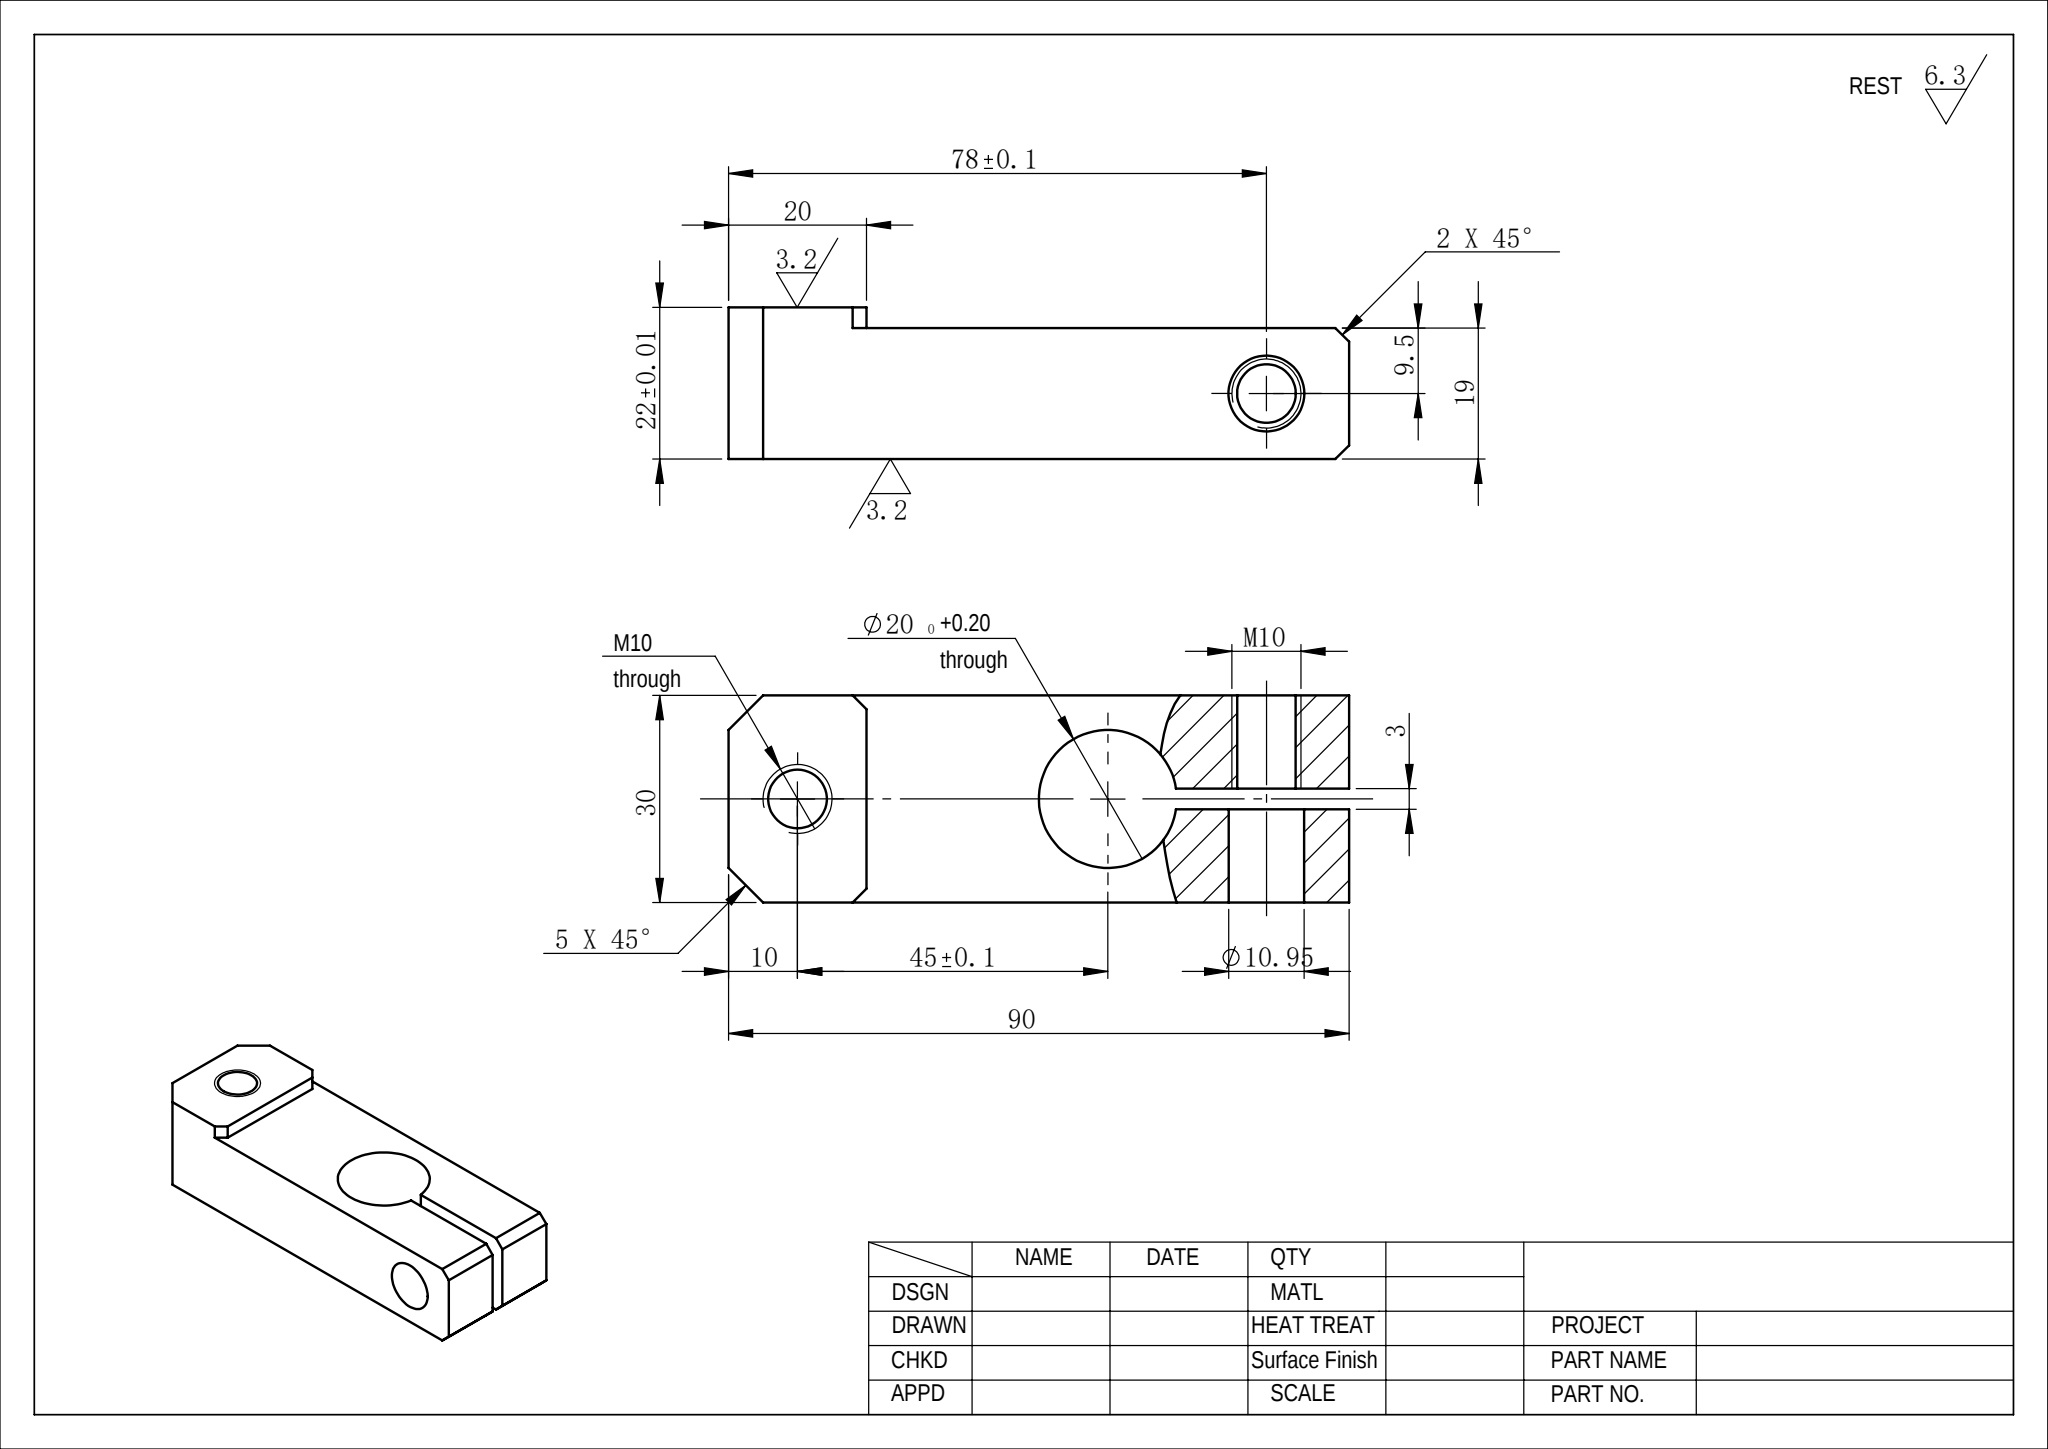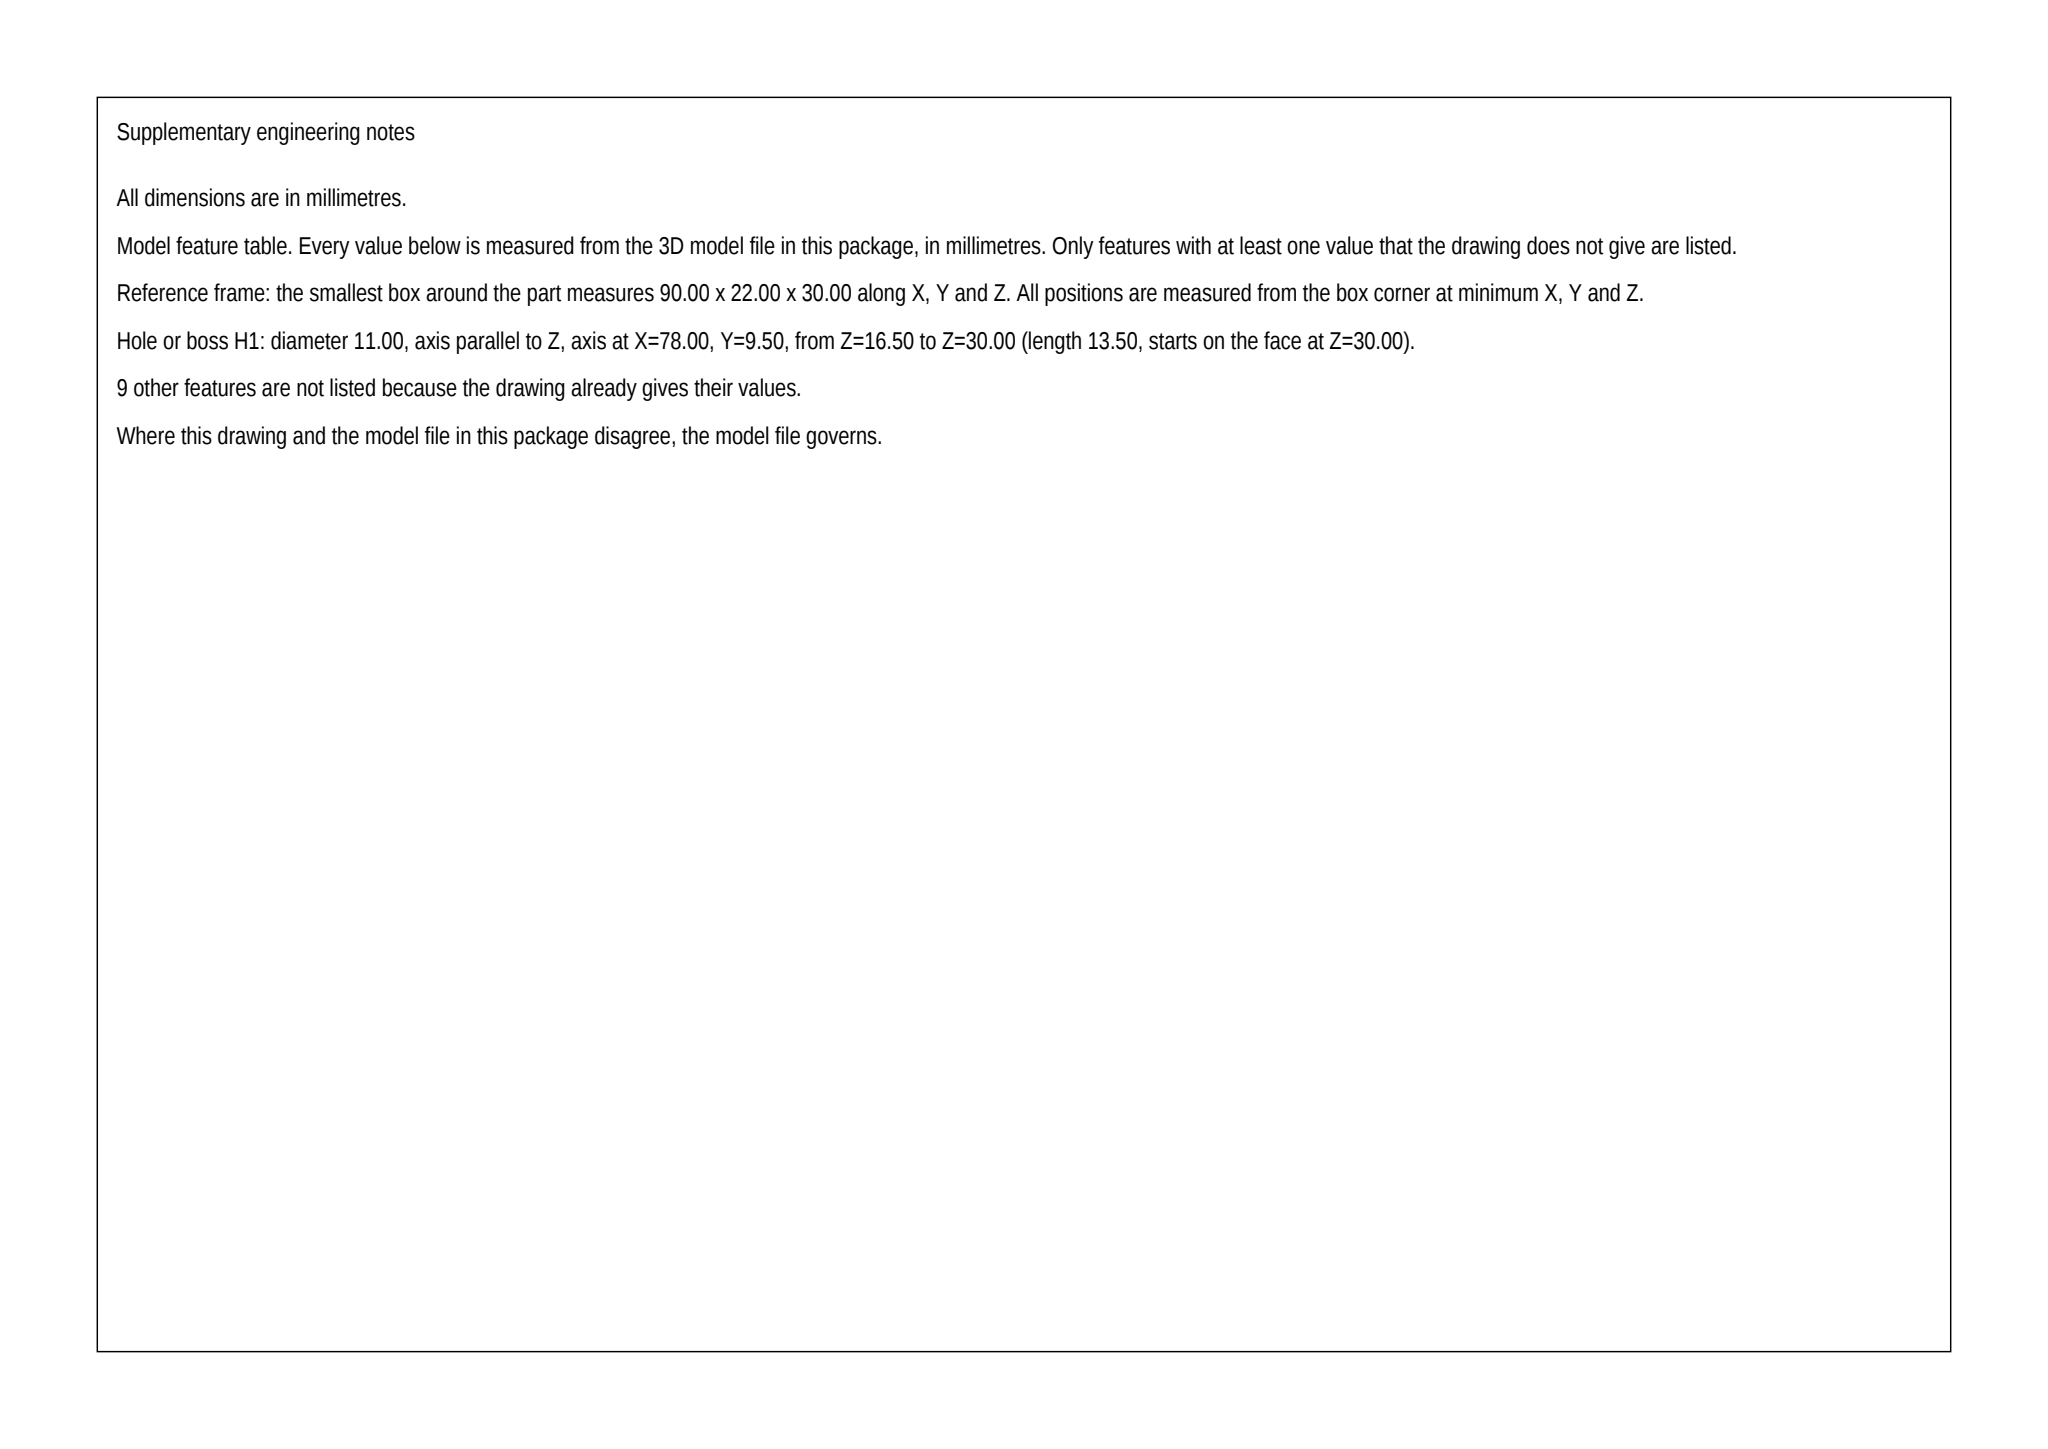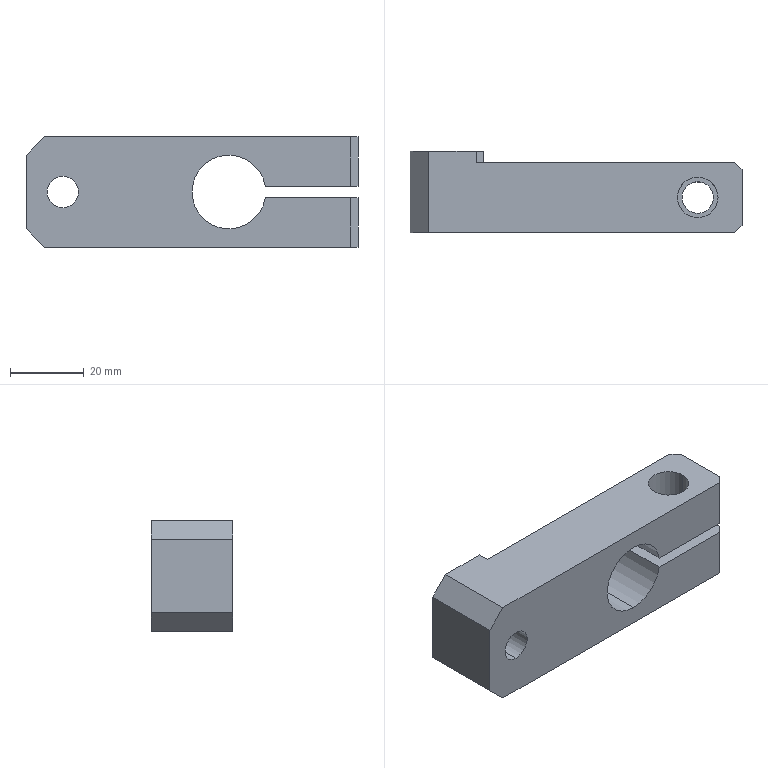Part | SolidWorks | mm | 1 solid | 28 faces | box 90 x 22 x 30 mm | volume 41736 mm3 | plane 19 | cylinder 9 | commonest cylinder face diameters 8.5 x4 20 x3 11 x2
build123d program:
from build123d import *

# Parameters (mm, degrees)
EXTRUDE1_DEPTH     = 30
M10_TAPPED_HOLE1_D = 8.5
SKETCH4_R          = 10
CUT_EXTRUDE1_DEPTH = 97.752
SKETCH5_R          = 5.5
CUT_EXTRUDE2_DEPTH = 15
SKETCH6_W          = 40.815
SKETCH6_H          = 3
CUT_EXTRUDE3_DEPTH = 97.752
M10_TAPPED_HOLE2_D = 8.5
CHAMFER1_SIZE      = 5
CHAMFER2_SIZE      = 2


with BuildPart() as part:
    # Sketch1 → Extrude1 (new body)
    with BuildSketch(Plane.XY):
        Polygon((0, 0), (0, 22), (20, 22), (20, 19), (90, 19), (90, 0), align=None)
    extrude(amount=EXTRUDE1_DEPTH)

    # M10 Tapped Hole1 (through all)
    with Locations(Plane(origin=(0, 22, 0), x_dir=(-1, 0, 0), z_dir=(0, 1, 0))):
        with Locations((-10, 15)):
            Hole(M10_TAPPED_HOLE1_D / 2)

    # Sketch4 → Cut-Extrude1 (cut, through all)
    with BuildSketch(Plane(origin=(0, 19, 0), x_dir=(1, 0, 0), z_dir=(0, 1, 0))):
        with Locations(Location((55, -15, 0), (0, 0, 270))):
            Circle(SKETCH4_R)
    extrude(amount=-CUT_EXTRUDE1_DEPTH, mode=Mode.SUBTRACT)

    # Sketch5 → Cut-Extrude2 (cut)
    with BuildSketch(Plane.XY.offset(30)):
        with Locations((78, 9.5)):
            Circle(SKETCH5_R)
    extrude(amount=-CUT_EXTRUDE2_DEPTH, mode=Mode.SUBTRACT)

    # Sketch6 → Cut-Extrude3 (cut, through all)
    with BuildSketch(Plane(origin=(0, 19, 0), x_dir=(1, 0, 0), z_dir=(0, 1, 0))):
        with Locations((72.3, -15)):
            Rectangle(SKETCH6_W, SKETCH6_H)
    extrude(amount=-CUT_EXTRUDE3_DEPTH, mode=Mode.SUBTRACT)

    # M10 Tapped Hole2 (through all)
    with Locations(Plane.XY.offset(13.5)):
        with Locations((78, 9.5)):
            Hole(M10_TAPPED_HOLE2_D / 2)

    # Chamfer1
    chamfer1_edges = [part.edges().sort_by_distance(p)[0] for p in [
        (0, 11, 30),
        (0, 11, 0),
    ]]
    chamfer(chamfer1_edges, length=CHAMFER1_SIZE)

    # Chamfer2
    chamfer2_edges = [part.edges().sort_by_distance(p)[0] for p in [
        (90, 19, 23.25),
        (90, 0, 23.25),
        (20, 20.5, 30),
        (90, 19, 6.75),
        (90, 0, 6.75),
        (20, 20.5, 0),
    ]]
    chamfer(chamfer2_edges, length=CHAMFER2_SIZE)


solid = part.part
STEP:
#1=CARTESIAN_POINT('',(73.75,9.5,0.));
#2=VERTEX_POINT('',#1);
#3=CARTESIAN_POINT('',(82.25,9.5,0.));
#4=VERTEX_POINT('',#3);
#5=CARTESIAN_POINT('',(78.,9.5,0.));
#6=DIRECTION('',(0.,0.,1.));
#7=DIRECTION('',(1.,0.,0.));
#8=AXIS2_PLACEMENT_3D('',#5,#6,#7);
#9=CIRCLE('',#8,4.25);
#10=EDGE_CURVE('',#2,#4,#9,.T.);
#11=ORIENTED_EDGE('',*,*,#10,.F.);
#12=CARTESIAN_POINT('',(73.75,9.5,13.5));
#13=VERTEX_POINT('',#12);
#14=CARTESIAN_POINT('',(73.75,9.5,13.5));
#15=DIRECTION('',(0.,0.,1.));
#16=VECTOR('',#15,1000.);
#17=LINE('',#14,#16);
#18=EDGE_CURVE('',#2,#13,#17,.T.);
#19=ORIENTED_EDGE('',*,*,#18,.T.);
#20=CARTESIAN_POINT('',(82.25,9.5,13.5));
#21=VERTEX_POINT('',#20);
#22=CARTESIAN_POINT('',(78.,9.5,13.5));
#23=DIRECTION('',(0.,0.,1.));
#24=DIRECTION('',(1.,0.,0.));
#25=AXIS2_PLACEMENT_3D('',#22,#23,#24);
#26=CIRCLE('',#25,4.25);
#27=EDGE_CURVE('',#13,#21,#26,.T.);
#28=ORIENTED_EDGE('',*,*,#27,.T.);
#29=CARTESIAN_POINT('',(82.25,9.5,13.5));
#30=DIRECTION('',(0.,0.,1.));
#31=VECTOR('',#30,1000.);
#32=LINE('',#29,#31);
#33=EDGE_CURVE('',#4,#21,#32,.T.);
#34=ORIENTED_EDGE('',*,*,#33,.F.);
#35=EDGE_LOOP('',(#11,#19,#28,#34));
#36=FACE_OUTER_BOUND('',#35,.T.);
#37=CARTESIAN_POINT('',(78.,9.5,13.5));
#38=DIRECTION('',(0.,0.,1.));
#39=DIRECTION('',(1.,0.,0.));
#40=AXIS2_PLACEMENT_3D('',#37,#38,#39);
#41=CYLINDRICAL_SURFACE('',#40,4.25);
#42=ADVANCED_FACE('',(#36),#41,.F.);
#43=CARTESIAN_POINT('',(83.5,9.5,16.5));
#44=VERTEX_POINT('',#43);
#45=CARTESIAN_POINT('',(72.5,9.5,16.5));
#46=VERTEX_POINT('',#45);
#47=CARTESIAN_POINT('',(78.,9.5,16.5));
#48=DIRECTION('',(0.,0.,-1.));
#49=DIRECTION('',(1.,0.,0.));
#50=AXIS2_PLACEMENT_3D('',#47,#48,#49);
#51=CIRCLE('',#50,5.5);
#52=EDGE_CURVE('',#44,#46,#51,.T.);
#53=ORIENTED_EDGE('',*,*,#52,.T.);
#54=CARTESIAN_POINT('',(72.5,9.5,30.));
#55=VERTEX_POINT('',#54);
#56=CARTESIAN_POINT('',(72.5,9.5,15.));
#57=DIRECTION('',(0.,0.,1.));
#58=VECTOR('',#57,1000.);
#59=LINE('',#56,#58);
#60=EDGE_CURVE('',#46,#55,#59,.T.);
#61=ORIENTED_EDGE('',*,*,#60,.T.);
#62=CARTESIAN_POINT('',(83.5,9.5,30.));
#63=VERTEX_POINT('',#62);
#64=CARTESIAN_POINT('',(78.,9.5,30.));
#65=DIRECTION('',(0.,0.,1.));
#66=DIRECTION('',(1.,0.,0.));
#67=AXIS2_PLACEMENT_3D('',#64,#65,#66);
#68=CIRCLE('',#67,5.5);
#69=EDGE_CURVE('',#55,#63,#68,.T.);
#70=ORIENTED_EDGE('',*,*,#69,.T.);
#71=CARTESIAN_POINT('',(83.5,9.5,15.));
#72=DIRECTION('',(0.,0.,1.));
#73=VECTOR('',#72,1000.);
#74=LINE('',#71,#73);
#75=EDGE_CURVE('',#44,#63,#74,.T.);
#76=ORIENTED_EDGE('',*,*,#75,.F.);
#77=EDGE_LOOP('',(#53,#61,#70,#76));
#78=FACE_OUTER_BOUND('',#77,.T.);
#79=CARTESIAN_POINT('',(78.,9.5,15.));
#80=DIRECTION('',(0.,0.,1.));
#81=DIRECTION('',(1.,0.,0.));
#82=AXIS2_PLACEMENT_3D('',#79,#80,#81);
#83=CYLINDRICAL_SURFACE('',#82,5.5);
#84=ADVANCED_FACE('',(#78),#83,.F.);
#85=CARTESIAN_POINT('',(55.,0.,5.));
#86=VERTEX_POINT('',#85);
#87=CARTESIAN_POINT('',(55.,0.,25.));
#88=VERTEX_POINT('',#87);
#89=CARTESIAN_POINT('',(55.,0.,15.));
#90=DIRECTION('',(0.,1.,0.));
#91=DIRECTION('',(0.,0.,1.));
#92=AXIS2_PLACEMENT_3D('',#89,#90,#91);
#93=CIRCLE('',#92,10.);
#94=EDGE_CURVE('',#86,#88,#93,.T.);
#95=ORIENTED_EDGE('',*,*,#94,.F.);
#96=CARTESIAN_POINT('',(55.,19.,5.));
#97=VERTEX_POINT('',#96);
#98=CARTESIAN_POINT('',(55.,0.,5.));
#99=DIRECTION('',(0.,1.,0.));
#100=VECTOR('',#99,1000.);
#101=LINE('',#98,#100);
#102=EDGE_CURVE('',#86,#97,#101,.T.);
#103=ORIENTED_EDGE('',*,*,#102,.T.);
#104=CARTESIAN_POINT('',(55.,19.,25.));
#105=VERTEX_POINT('',#104);
#106=CARTESIAN_POINT('',(55.,19.,15.));
#107=DIRECTION('',(0.,1.,0.));
#108=DIRECTION('',(0.,0.,1.));
#109=AXIS2_PLACEMENT_3D('',#106,#107,#108);
#110=CIRCLE('',#109,10.);
#111=EDGE_CURVE('',#97,#105,#110,.T.);
#112=ORIENTED_EDGE('',*,*,#111,.T.);
#113=CARTESIAN_POINT('',(55.,0.,25.));
#114=DIRECTION('',(0.,1.,0.));
#115=VECTOR('',#114,1000.);
#116=LINE('',#113,#115);
#117=EDGE_CURVE('',#88,#105,#116,.T.);
#118=ORIENTED_EDGE('',*,*,#117,.F.);
#119=EDGE_LOOP('',(#95,#103,#112,#118));
#120=FACE_OUTER_BOUND('',#119,.T.);
#121=CARTESIAN_POINT('',(55.,0.,15.));
#122=DIRECTION('',(0.,1.,0.));
#123=DIRECTION('',(0.,0.,1.));
#124=AXIS2_PLACEMENT_3D('',#121,#122,#123);
#125=CYLINDRICAL_SURFACE('',#124,10.);
#126=ADVANCED_FACE('',(#120),#125,.F.);
#127=CARTESIAN_POINT('',(64.887,0.,16.5));
#128=VERTEX_POINT('',#127);
#129=CARTESIAN_POINT('',(55.,0.,15.));
#130=DIRECTION('',(0.,1.,0.));
#131=DIRECTION('',(0.,0.,1.));
#132=AXIS2_PLACEMENT_3D('',#129,#130,#131);
#133=CIRCLE('',#132,10.);
#134=EDGE_CURVE('',#88,#128,#133,.T.);
#135=ORIENTED_EDGE('',*,*,#134,.F.);
#136=ORIENTED_EDGE('',*,*,#117,.T.);
#137=CARTESIAN_POINT('',(64.887,19.,16.5));
#138=VERTEX_POINT('',#137);
#139=CARTESIAN_POINT('',(55.,19.,15.));
#140=DIRECTION('',(0.,1.,0.));
#141=DIRECTION('',(0.,0.,1.));
#142=AXIS2_PLACEMENT_3D('',#139,#140,#141);
#143=CIRCLE('',#142,10.);
#144=EDGE_CURVE('',#105,#138,#143,.T.);
#145=ORIENTED_EDGE('',*,*,#144,.T.);
#146=CARTESIAN_POINT('',(64.887,0.,16.5));
#147=DIRECTION('',(0.,-1.,0.));
#148=VECTOR('',#147,1000.);
#149=LINE('',#146,#148);
#150=EDGE_CURVE('',#138,#128,#149,.T.);
#151=ORIENTED_EDGE('',*,*,#150,.T.);
#152=EDGE_LOOP('',(#135,#136,#145,#151));
#153=FACE_OUTER_BOUND('',#152,.T.);
#154=CARTESIAN_POINT('',(55.,0.,15.));
#155=DIRECTION('',(0.,1.,0.));
#156=DIRECTION('',(0.,0.,1.));
#157=AXIS2_PLACEMENT_3D('',#154,#155,#156);
#158=CYLINDRICAL_SURFACE('',#157,10.);
#159=ADVANCED_FACE('',(#153),#158,.F.);
#160=CARTESIAN_POINT('',(10.,0.,10.75));
#161=VERTEX_POINT('',#160);
#162=CARTESIAN_POINT('',(10.,0.,19.25));
#163=VERTEX_POINT('',#162);
#164=CARTESIAN_POINT('',(10.,0.,15.));
#165=DIRECTION('',(0.,1.,0.));
#166=DIRECTION('',(0.,0.,1.));
#167=AXIS2_PLACEMENT_3D('',#164,#165,#166);
#168=CIRCLE('',#167,4.25);
#169=EDGE_CURVE('',#161,#163,#168,.T.);
#170=ORIENTED_EDGE('',*,*,#169,.F.);
#171=CARTESIAN_POINT('',(10.,22.,10.75));
#172=VERTEX_POINT('',#171);
#173=CARTESIAN_POINT('',(10.,22.,10.75));
#174=DIRECTION('',(0.,1.,0.));
#175=VECTOR('',#174,1000.);
#176=LINE('',#173,#175);
#177=EDGE_CURVE('',#161,#172,#176,.T.);
#178=ORIENTED_EDGE('',*,*,#177,.T.);
#179=CARTESIAN_POINT('',(10.,22.,19.25));
#180=VERTEX_POINT('',#179);
#181=CARTESIAN_POINT('',(10.,22.,15.));
#182=DIRECTION('',(0.,1.,0.));
#183=DIRECTION('',(0.,0.,1.));
#184=AXIS2_PLACEMENT_3D('',#181,#182,#183);
#185=CIRCLE('',#184,4.25);
#186=EDGE_CURVE('',#172,#180,#185,.T.);
#187=ORIENTED_EDGE('',*,*,#186,.T.);
#188=CARTESIAN_POINT('',(10.,22.,19.25));
#189=DIRECTION('',(0.,1.,0.));
#190=VECTOR('',#189,1000.);
#191=LINE('',#188,#190);
#192=EDGE_CURVE('',#163,#180,#191,.T.);
#193=ORIENTED_EDGE('',*,*,#192,.F.);
#194=EDGE_LOOP('',(#170,#178,#187,#193));
#195=FACE_OUTER_BOUND('',#194,.T.);
#196=CARTESIAN_POINT('',(10.,22.,15.));
#197=DIRECTION('',(0.,1.,0.));
#198=DIRECTION('',(0.,0.,1.));
#199=AXIS2_PLACEMENT_3D('',#196,#197,#198);
#200=CYLINDRICAL_SURFACE('',#199,4.25);
#201=ADVANCED_FACE('',(#195),#200,.F.);
#202=CARTESIAN_POINT('',(18.,22.,0.));
#203=VERTEX_POINT('',#202);
#204=CARTESIAN_POINT('',(5.,22.,-0.));
#205=VERTEX_POINT('',#204);
#206=CARTESIAN_POINT('',(0.,22.,0.));
#207=DIRECTION('',(-1.,0.,0.));
#208=VECTOR('',#207,1000.);
#209=LINE('',#206,#208);
#210=EDGE_CURVE('',#203,#205,#209,.T.);
#211=ORIENTED_EDGE('',*,*,#210,.F.);
#212=CARTESIAN_POINT('',(18.,19.,0.));
#213=VERTEX_POINT('',#212);
#214=CARTESIAN_POINT('',(18.,19.,0.));
#215=DIRECTION('',(0.,-1.,0.));
#216=VECTOR('',#215,1000.);
#217=LINE('',#214,#216);
#218=EDGE_CURVE('',#203,#213,#217,.T.);
#219=ORIENTED_EDGE('',*,*,#218,.T.);
#220=CARTESIAN_POINT('',(88.,19.,0.));
#221=VERTEX_POINT('',#220);
#222=CARTESIAN_POINT('',(20.,19.,0.));
#223=DIRECTION('',(-1.,0.,0.));
#224=VECTOR('',#223,1000.);
#225=LINE('',#222,#224);
#226=EDGE_CURVE('',#221,#213,#225,.T.);
#227=ORIENTED_EDGE('',*,*,#226,.F.);
#228=CARTESIAN_POINT('',(90.,17.,0.));
#229=VERTEX_POINT('',#228);
#230=CARTESIAN_POINT('',(53.5,53.5,0.));
#231=DIRECTION('',(0.7071,-0.7071,0.));
#232=VECTOR('',#231,1000.);
#233=LINE('',#230,#232);
#234=EDGE_CURVE('',#221,#229,#233,.T.);
#235=ORIENTED_EDGE('',*,*,#234,.T.);
#236=CARTESIAN_POINT('',(90.,2.,0.));
#237=VERTEX_POINT('',#236);
#238=CARTESIAN_POINT('',(90.,19.,0.));
#239=DIRECTION('',(0.,1.,0.));
#240=VECTOR('',#239,1000.);
#241=LINE('',#238,#240);
#242=EDGE_CURVE('',#237,#229,#241,.T.);
#243=ORIENTED_EDGE('',*,*,#242,.F.);
#244=CARTESIAN_POINT('',(88.,0.,0.));
#245=VERTEX_POINT('',#244);
#246=CARTESIAN_POINT('',(44.,-44.,0.));
#247=DIRECTION('',(-0.7071,-0.7071,0.));
#248=VECTOR('',#247,1000.);
#249=LINE('',#246,#248);
#250=EDGE_CURVE('',#237,#245,#249,.T.);
#251=ORIENTED_EDGE('',*,*,#250,.T.);
#252=CARTESIAN_POINT('',(5.,0.,0.));
#253=VERTEX_POINT('',#252);
#254=CARTESIAN_POINT('',(90.,0.,0.));
#255=DIRECTION('',(1.,0.,0.));
#256=VECTOR('',#255,1000.);
#257=LINE('',#254,#256);
#258=EDGE_CURVE('',#253,#245,#257,.T.);
#259=ORIENTED_EDGE('',*,*,#258,.F.);
#260=CARTESIAN_POINT('',(5.,22.,0.));
#261=DIRECTION('',(0.,1.,0.));
#262=VECTOR('',#261,1000.);
#263=LINE('',#260,#262);
#264=EDGE_CURVE('',#253,#205,#263,.T.);
#265=ORIENTED_EDGE('',*,*,#264,.T.);
#266=EDGE_LOOP('',(#211,#219,#227,#235,#243,#251,#259,#265));
#267=FACE_OUTER_BOUND('',#266,.T.);
#268=CARTESIAN_POINT('',(78.,9.5,0.));
#269=DIRECTION('',(0.,0.,1.));
#270=DIRECTION('',(1.,0.,0.));
#271=AXIS2_PLACEMENT_3D('',#268,#269,#270);
#272=CIRCLE('',#271,4.25);
#273=EDGE_CURVE('',#4,#2,#272,.T.);
#274=ORIENTED_EDGE('',*,*,#273,.T.);
#275=ORIENTED_EDGE('',*,*,#10,.T.);
#276=EDGE_LOOP('',(#274,#275));
#277=FACE_BOUND('',#276,.T.);
#278=CARTESIAN_POINT('',(0.,0.,0.));
#279=DIRECTION('',(0.,0.,-1.));
#280=DIRECTION('',(-1.,0.,0.));
#281=AXIS2_PLACEMENT_3D('',#278,#279,#280);
#282=PLANE('',#281);
#283=ADVANCED_FACE('',(#267,#277),#282,.T.);
#284=CARTESIAN_POINT('',(90.,17.,13.5));
#285=VERTEX_POINT('',#284);
#286=CARTESIAN_POINT('',(90.,2.,13.5));
#287=VERTEX_POINT('',#286);
#288=CARTESIAN_POINT('',(90.,19.,13.5));
#289=DIRECTION('',(0.,-1.,0.));
#290=VECTOR('',#289,1000.);
#291=LINE('',#288,#290);
#292=EDGE_CURVE('',#285,#287,#291,.T.);
#293=ORIENTED_EDGE('',*,*,#292,.T.);
#294=CARTESIAN_POINT('',(90.,2.,30.));
#295=DIRECTION('',(0.,0.,-1.));
#296=VECTOR('',#295,1000.);
#297=LINE('',#294,#296);
#298=EDGE_CURVE('',#287,#237,#297,.T.);
#299=ORIENTED_EDGE('',*,*,#298,.T.);
#300=ORIENTED_EDGE('',*,*,#242,.T.);
#301=CARTESIAN_POINT('',(90.,17.,30.));
#302=DIRECTION('',(0.,0.,1.));
#303=VECTOR('',#302,1000.);
#304=LINE('',#301,#303);
#305=EDGE_CURVE('',#229,#285,#304,.T.);
#306=ORIENTED_EDGE('',*,*,#305,.T.);
#307=EDGE_LOOP('',(#293,#299,#300,#306));
#308=FACE_OUTER_BOUND('',#307,.T.);
#309=CARTESIAN_POINT('',(90.,19.,30.));
#310=DIRECTION('',(-1.,0.,0.));
#311=DIRECTION('',(0.,0.,1.));
#312=AXIS2_PLACEMENT_3D('',#309,#310,#311);
#313=PLANE('',#312);
#314=ADVANCED_FACE('',(#308),#313,.F.);
#315=ORIENTED_EDGE('',*,*,#258,.T.);
#316=CARTESIAN_POINT('',(88.,-0.,13.5));
#317=VERTEX_POINT('',#316);
#318=CARTESIAN_POINT('',(88.,0.,30.));
#319=DIRECTION('',(0.,0.,1.));
#320=VECTOR('',#319,1000.);
#321=LINE('',#318,#320);
#322=EDGE_CURVE('',#245,#317,#321,.T.);
#323=ORIENTED_EDGE('',*,*,#322,.T.);
#324=CARTESIAN_POINT('',(64.887,0.,13.5));
#325=VERTEX_POINT('',#324);
#326=CARTESIAN_POINT('',(51.893,0.,13.5));
#327=DIRECTION('',(-1.,0.,0.));
#328=VECTOR('',#327,1000.);
#329=LINE('',#326,#328);
#330=EDGE_CURVE('',#317,#325,#329,.T.);
#331=ORIENTED_EDGE('',*,*,#330,.T.);
#332=CARTESIAN_POINT('',(55.,0.,15.));
#333=DIRECTION('',(0.,1.,0.));
#334=DIRECTION('',(0.,0.,1.));
#335=AXIS2_PLACEMENT_3D('',#332,#333,#334);
#336=CIRCLE('',#335,10.);
#337=EDGE_CURVE('',#325,#86,#336,.T.);
#338=ORIENTED_EDGE('',*,*,#337,.T.);
#339=ORIENTED_EDGE('',*,*,#94,.T.);
#340=ORIENTED_EDGE('',*,*,#134,.T.);
#341=CARTESIAN_POINT('',(88.,0.,16.5));
#342=VERTEX_POINT('',#341);
#343=CARTESIAN_POINT('',(51.893,0.,16.5));
#344=DIRECTION('',(1.,0.,0.));
#345=VECTOR('',#344,1000.);
#346=LINE('',#343,#345);
#347=EDGE_CURVE('',#128,#342,#346,.T.);
#348=ORIENTED_EDGE('',*,*,#347,.T.);
#349=CARTESIAN_POINT('',(88.,0.,30.));
#350=VERTEX_POINT('',#349);
#351=CARTESIAN_POINT('',(88.,0.,30.));
#352=DIRECTION('',(0.,0.,1.));
#353=VECTOR('',#352,1000.);
#354=LINE('',#351,#353);
#355=EDGE_CURVE('',#342,#350,#354,.T.);
#356=ORIENTED_EDGE('',*,*,#355,.T.);
#357=CARTESIAN_POINT('',(5.,0.,30.));
#358=VERTEX_POINT('',#357);
#359=CARTESIAN_POINT('',(90.,0.,30.));
#360=DIRECTION('',(1.,0.,0.));
#361=VECTOR('',#360,1000.);
#362=LINE('',#359,#361);
#363=EDGE_CURVE('',#358,#350,#362,.T.);
#364=ORIENTED_EDGE('',*,*,#363,.F.);
#365=CARTESIAN_POINT('',(0.,0.,25.));
#366=VERTEX_POINT('',#365);
#367=CARTESIAN_POINT('',(5.,0.,30.));
#368=DIRECTION('',(-0.7071,-0.,-0.7071));
#369=VECTOR('',#368,1000.);
#370=LINE('',#367,#369);
#371=EDGE_CURVE('',#358,#366,#370,.T.);
#372=ORIENTED_EDGE('',*,*,#371,.T.);
#373=CARTESIAN_POINT('',(0.,0.,5.));
#374=VERTEX_POINT('',#373);
#375=CARTESIAN_POINT('',(0.,0.,30.));
#376=DIRECTION('',(0.,0.,-1.));
#377=VECTOR('',#376,1000.);
#378=LINE('',#375,#377);
#379=EDGE_CURVE('',#366,#374,#378,.T.);
#380=ORIENTED_EDGE('',*,*,#379,.T.);
#381=CARTESIAN_POINT('',(0.,0.,5.));
#382=DIRECTION('',(0.7071,0.,-0.7071));
#383=VECTOR('',#382,1000.);
#384=LINE('',#381,#383);
#385=EDGE_CURVE('',#374,#253,#384,.T.);
#386=ORIENTED_EDGE('',*,*,#385,.T.);
#387=EDGE_LOOP('',(#315,#323,#331,#338,#339,#340,#348,#356,#364,#372,#380,#386));
#388=FACE_OUTER_BOUND('',#387,.T.);
#389=CARTESIAN_POINT('',(10.,0.,15.));
#390=DIRECTION('',(0.,1.,0.));
#391=DIRECTION('',(0.,0.,1.));
#392=AXIS2_PLACEMENT_3D('',#389,#390,#391);
#393=CIRCLE('',#392,4.25);
#394=EDGE_CURVE('',#163,#161,#393,.T.);
#395=ORIENTED_EDGE('',*,*,#394,.T.);
#396=ORIENTED_EDGE('',*,*,#169,.T.);
#397=EDGE_LOOP('',(#395,#396));
#398=FACE_BOUND('',#397,.T.);
#399=CARTESIAN_POINT('',(90.,0.,30.));
#400=DIRECTION('',(-0.,1.,0.));
#401=DIRECTION('',(-1.,-0.,0.));
#402=AXIS2_PLACEMENT_3D('',#399,#400,#401);
#403=PLANE('',#402);
#404=ADVANCED_FACE('',(#388,#398),#403,.F.);
#405=CARTESIAN_POINT('',(90.,2.,30.));
#406=VERTEX_POINT('',#405);
#407=CARTESIAN_POINT('',(90.,17.,30.));
#408=VERTEX_POINT('',#407);
#409=CARTESIAN_POINT('',(90.,19.,30.));
#410=DIRECTION('',(0.,1.,0.));
#411=VECTOR('',#410,1000.);
#412=LINE('',#409,#411);
#413=EDGE_CURVE('',#406,#408,#412,.T.);
#414=ORIENTED_EDGE('',*,*,#413,.F.);
#415=CARTESIAN_POINT('',(90.,2.,16.5));
#416=VERTEX_POINT('',#415);
#417=CARTESIAN_POINT('',(90.,2.,30.));
#418=DIRECTION('',(0.,0.,-1.));
#419=VECTOR('',#418,1000.);
#420=LINE('',#417,#419);
#421=EDGE_CURVE('',#406,#416,#420,.T.);
#422=ORIENTED_EDGE('',*,*,#421,.T.);
#423=CARTESIAN_POINT('',(90.,17.,16.5));
#424=VERTEX_POINT('',#423);
#425=CARTESIAN_POINT('',(90.,19.,16.5));
#426=DIRECTION('',(0.,1.,0.));
#427=VECTOR('',#426,1000.);
#428=LINE('',#425,#427);
#429=EDGE_CURVE('',#416,#424,#428,.T.);
#430=ORIENTED_EDGE('',*,*,#429,.T.);
#431=CARTESIAN_POINT('',(90.,17.,30.));
#432=DIRECTION('',(0.,0.,1.));
#433=VECTOR('',#432,1000.);
#434=LINE('',#431,#433);
#435=EDGE_CURVE('',#424,#408,#434,.T.);
#436=ORIENTED_EDGE('',*,*,#435,.T.);
#437=EDGE_LOOP('',(#414,#422,#430,#436));
#438=FACE_OUTER_BOUND('',#437,.T.);
#439=CARTESIAN_POINT('',(90.,19.,30.));
#440=DIRECTION('',(-1.,0.,0.));
#441=DIRECTION('',(0.,0.,1.));
#442=AXIS2_PLACEMENT_3D('',#439,#440,#441);
#443=PLANE('',#442);
#444=ADVANCED_FACE('',(#438),#443,.F.);
#445=CARTESIAN_POINT('',(88.,19.,13.5));
#446=VERTEX_POINT('',#445);
#447=CARTESIAN_POINT('',(64.887,19.,13.5));
#448=VERTEX_POINT('',#447);
#449=CARTESIAN_POINT('',(51.893,19.,13.5));
#450=DIRECTION('',(-1.,0.,0.));
#451=VECTOR('',#450,1000.);
#452=LINE('',#449,#451);
#453=EDGE_CURVE('',#446,#448,#452,.T.);
#454=ORIENTED_EDGE('',*,*,#453,.F.);
#455=CARTESIAN_POINT('',(88.,19.,30.));
#456=DIRECTION('',(0.,0.,-1.));
#457=VECTOR('',#456,1000.);
#458=LINE('',#455,#457);
#459=EDGE_CURVE('',#446,#221,#458,.T.);
#460=ORIENTED_EDGE('',*,*,#459,.T.);
#461=ORIENTED_EDGE('',*,*,#226,.T.);
#462=CARTESIAN_POINT('',(20.,19.,2.));
#463=VERTEX_POINT('',#462);
#464=CARTESIAN_POINT('',(34.,19.,16.));
#465=DIRECTION('',(0.7071,0.,0.7071));
#466=VECTOR('',#465,1000.);
#467=LINE('',#464,#466);
#468=EDGE_CURVE('',#213,#463,#467,.T.);
#469=ORIENTED_EDGE('',*,*,#468,.T.);
#470=CARTESIAN_POINT('',(20.,19.,28.));
#471=VERTEX_POINT('',#470);
#472=CARTESIAN_POINT('',(20.,19.,30.));
#473=DIRECTION('',(0.,0.,-1.));
#474=VECTOR('',#473,1000.);
#475=LINE('',#472,#474);
#476=EDGE_CURVE('',#471,#463,#475,.T.);
#477=ORIENTED_EDGE('',*,*,#476,.F.);
#478=CARTESIAN_POINT('',(18.,19.,30.));
#479=VERTEX_POINT('',#478);
#480=CARTESIAN_POINT('',(19.,19.,29.));
#481=DIRECTION('',(-0.7071,0.,0.7071));
#482=VECTOR('',#481,1000.);
#483=LINE('',#480,#482);
#484=EDGE_CURVE('',#471,#479,#483,.T.);
#485=ORIENTED_EDGE('',*,*,#484,.T.);
#486=CARTESIAN_POINT('',(88.,19.,30.));
#487=VERTEX_POINT('',#486);
#488=CARTESIAN_POINT('',(20.,19.,30.));
#489=DIRECTION('',(-1.,0.,0.));
#490=VECTOR('',#489,1000.);
#491=LINE('',#488,#490);
#492=EDGE_CURVE('',#487,#479,#491,.T.);
#493=ORIENTED_EDGE('',*,*,#492,.F.);
#494=CARTESIAN_POINT('',(88.,19.,16.5));
#495=VERTEX_POINT('',#494);
#496=CARTESIAN_POINT('',(88.,19.,30.));
#497=DIRECTION('',(0.,0.,-1.));
#498=VECTOR('',#497,1000.);
#499=LINE('',#496,#498);
#500=EDGE_CURVE('',#487,#495,#499,.T.);
#501=ORIENTED_EDGE('',*,*,#500,.T.);
#502=CARTESIAN_POINT('',(51.893,19.,16.5));
#503=DIRECTION('',(1.,0.,0.));
#504=VECTOR('',#503,1000.);
#505=LINE('',#502,#504);
#506=EDGE_CURVE('',#138,#495,#505,.T.);
#507=ORIENTED_EDGE('',*,*,#506,.F.);
#508=ORIENTED_EDGE('',*,*,#144,.F.);
#509=ORIENTED_EDGE('',*,*,#111,.F.);
#510=CARTESIAN_POINT('',(55.,19.,15.));
#511=DIRECTION('',(0.,1.,0.));
#512=DIRECTION('',(0.,0.,1.));
#513=AXIS2_PLACEMENT_3D('',#510,#511,#512);
#514=CIRCLE('',#513,10.);
#515=EDGE_CURVE('',#448,#97,#514,.T.);
#516=ORIENTED_EDGE('',*,*,#515,.F.);
#517=EDGE_LOOP('',(#454,#460,#461,#469,#477,#485,#493,#501,#507,#508,#509,#516));
#518=FACE_OUTER_BOUND('',#517,.T.);
#519=CARTESIAN_POINT('',(20.,19.,30.));
#520=DIRECTION('',(0.,-1.,0.));
#521=DIRECTION('',(0.,0.,-1.));
#522=AXIS2_PLACEMENT_3D('',#519,#520,#521);
#523=PLANE('',#522);
#524=ADVANCED_FACE('',(#518),#523,.F.);
#525=ORIENTED_EDGE('',*,*,#476,.T.);
#526=CARTESIAN_POINT('',(20.,22.,2.));
#527=VERTEX_POINT('',#526);
#528=CARTESIAN_POINT('',(20.,22.,2.));
#529=DIRECTION('',(0.,1.,0.));
#530=VECTOR('',#529,1000.);
#531=LINE('',#528,#530);
#532=EDGE_CURVE('',#463,#527,#531,.T.);
#533=ORIENTED_EDGE('',*,*,#532,.T.);
#534=CARTESIAN_POINT('',(20.,22.,28.));
#535=VERTEX_POINT('',#534);
#536=CARTESIAN_POINT('',(20.,22.,30.));
#537=DIRECTION('',(0.,0.,-1.));
#538=VECTOR('',#537,1000.);
#539=LINE('',#536,#538);
#540=EDGE_CURVE('',#535,#527,#539,.T.);
#541=ORIENTED_EDGE('',*,*,#540,.F.);
#542=CARTESIAN_POINT('',(20.,22.,28.));
#543=DIRECTION('',(0.,-1.,0.));
#544=VECTOR('',#543,1000.);
#545=LINE('',#542,#544);
#546=EDGE_CURVE('',#535,#471,#545,.T.);
#547=ORIENTED_EDGE('',*,*,#546,.T.);
#548=EDGE_LOOP('',(#525,#533,#541,#547));
#549=FACE_OUTER_BOUND('',#548,.T.);
#550=CARTESIAN_POINT('',(20.,22.,30.));
#551=DIRECTION('',(-1.,0.,0.));
#552=DIRECTION('',(0.,0.,1.));
#553=AXIS2_PLACEMENT_3D('',#550,#551,#552);
#554=PLANE('',#553);
#555=ADVANCED_FACE('',(#549),#554,.F.);
#556=CARTESIAN_POINT('',(10.,22.,15.));
#557=DIRECTION('',(0.,1.,0.));
#558=DIRECTION('',(0.,0.,1.));
#559=AXIS2_PLACEMENT_3D('',#556,#557,#558);
#560=CIRCLE('',#559,4.25);
#561=EDGE_CURVE('',#180,#172,#560,.T.);
#562=ORIENTED_EDGE('',*,*,#561,.F.);
#563=ORIENTED_EDGE('',*,*,#186,.F.);
#564=EDGE_LOOP('',(#562,#563));
#565=FACE_BOUND('',#564,.T.);
#566=ORIENTED_EDGE('',*,*,#540,.T.);
#567=CARTESIAN_POINT('',(20.,22.,2.));
#568=DIRECTION('',(-0.7071,0.,-0.7071));
#569=VECTOR('',#568,1000.);
#570=LINE('',#567,#569);
#571=EDGE_CURVE('',#527,#203,#570,.T.);
#572=ORIENTED_EDGE('',*,*,#571,.T.);
#573=ORIENTED_EDGE('',*,*,#210,.T.);
#574=CARTESIAN_POINT('',(-0.,22.,5.));
#575=VERTEX_POINT('',#574);
#576=CARTESIAN_POINT('',(0.,22.,5.));
#577=DIRECTION('',(-0.7071,0.,0.7071));
#578=VECTOR('',#577,1000.);
#579=LINE('',#576,#578);
#580=EDGE_CURVE('',#205,#575,#579,.T.);
#581=ORIENTED_EDGE('',*,*,#580,.T.);
#582=CARTESIAN_POINT('',(0.,22.,25.));
#583=VERTEX_POINT('',#582);
#584=CARTESIAN_POINT('',(0.,22.,30.));
#585=DIRECTION('',(0.,0.,-1.));
#586=VECTOR('',#585,1000.);
#587=LINE('',#584,#586);
#588=EDGE_CURVE('',#583,#575,#587,.T.);
#589=ORIENTED_EDGE('',*,*,#588,.F.);
#590=CARTESIAN_POINT('',(5.,22.,30.));
#591=VERTEX_POINT('',#590);
#592=CARTESIAN_POINT('',(5.,22.,30.));
#593=DIRECTION('',(0.7071,0.,0.7071));
#594=VECTOR('',#593,1000.);
#595=LINE('',#592,#594);
#596=EDGE_CURVE('',#583,#591,#595,.T.);
#597=ORIENTED_EDGE('',*,*,#596,.T.);
#598=CARTESIAN_POINT('',(18.,22.,30.));
#599=VERTEX_POINT('',#598);
#600=CARTESIAN_POINT('',(0.,22.,30.));
#601=DIRECTION('',(-1.,0.,0.));
#602=VECTOR('',#601,1000.);
#603=LINE('',#600,#602);
#604=EDGE_CURVE('',#599,#591,#603,.T.);
#605=ORIENTED_EDGE('',*,*,#604,.F.);
#606=CARTESIAN_POINT('',(18.,22.,30.));
#607=DIRECTION('',(0.7071,0.,-0.7071));
#608=VECTOR('',#607,1000.);
#609=LINE('',#606,#608);
#610=EDGE_CURVE('',#599,#535,#609,.T.);
#611=ORIENTED_EDGE('',*,*,#610,.T.);
#612=EDGE_LOOP('',(#566,#572,#573,#581,#589,#597,#605,#611));
#613=FACE_OUTER_BOUND('',#612,.T.);
#614=CARTESIAN_POINT('',(0.,22.,30.));
#615=DIRECTION('',(0.,-1.,0.));
#616=DIRECTION('',(0.,0.,-1.));
#617=AXIS2_PLACEMENT_3D('',#614,#615,#616);
#618=PLANE('',#617);
#619=ADVANCED_FACE('',(#565,#613),#618,.F.);
#620=ORIENTED_EDGE('',*,*,#588,.T.);
#621=CARTESIAN_POINT('',(0.,0.,5.));
#622=DIRECTION('',(0.,-1.,0.));
#623=VECTOR('',#622,1000.);
#624=LINE('',#621,#623);
#625=EDGE_CURVE('',#575,#374,#624,.T.);
#626=ORIENTED_EDGE('',*,*,#625,.T.);
#627=ORIENTED_EDGE('',*,*,#379,.F.);
#628=CARTESIAN_POINT('',(0.,0.,25.));
#629=DIRECTION('',(0.,1.,0.));
#630=VECTOR('',#629,1000.);
#631=LINE('',#628,#630);
#632=EDGE_CURVE('',#366,#583,#631,.T.);
#633=ORIENTED_EDGE('',*,*,#632,.T.);
#634=EDGE_LOOP('',(#620,#626,#627,#633));
#635=FACE_OUTER_BOUND('',#634,.T.);
#636=CARTESIAN_POINT('',(0.,0.,30.));
#637=DIRECTION('',(1.,0.,0.));
#638=DIRECTION('',(0.,0.,-1.));
#639=AXIS2_PLACEMENT_3D('',#636,#637,#638);
#640=PLANE('',#639);
#641=ADVANCED_FACE('',(#635),#640,.F.);
#642=CARTESIAN_POINT('',(78.,9.5,30.));
#643=DIRECTION('',(0.,0.,1.));
#644=DIRECTION('',(1.,0.,0.));
#645=AXIS2_PLACEMENT_3D('',#642,#643,#644);
#646=CIRCLE('',#645,5.5);
#647=EDGE_CURVE('',#63,#55,#646,.T.);
#648=ORIENTED_EDGE('',*,*,#647,.F.);
#649=ORIENTED_EDGE('',*,*,#69,.F.);
#650=EDGE_LOOP('',(#648,#649));
#651=FACE_BOUND('',#650,.T.);
#652=ORIENTED_EDGE('',*,*,#492,.T.);
#653=CARTESIAN_POINT('',(18.,0.,30.));
#654=DIRECTION('',(0.,1.,0.));
#655=VECTOR('',#654,1000.);
#656=LINE('',#653,#655);
#657=EDGE_CURVE('',#479,#599,#656,.T.);
#658=ORIENTED_EDGE('',*,*,#657,.T.);
#659=ORIENTED_EDGE('',*,*,#604,.T.);
#660=CARTESIAN_POINT('',(5.,0.,30.));
#661=DIRECTION('',(0.,-1.,0.));
#662=VECTOR('',#661,1000.);
#663=LINE('',#660,#662);
#664=EDGE_CURVE('',#591,#358,#663,.T.);
#665=ORIENTED_EDGE('',*,*,#664,.T.);
#666=ORIENTED_EDGE('',*,*,#363,.T.);
#667=CARTESIAN_POINT('',(90.,2.,30.));
#668=DIRECTION('',(0.7071,0.7071,0.));
#669=VECTOR('',#668,1000.);
#670=LINE('',#667,#669);
#671=EDGE_CURVE('',#350,#406,#670,.T.);
#672=ORIENTED_EDGE('',*,*,#671,.T.);
#673=ORIENTED_EDGE('',*,*,#413,.T.);
#674=CARTESIAN_POINT('',(88.,19.,30.));
#675=DIRECTION('',(-0.7071,0.7071,0.));
#676=VECTOR('',#675,1000.);
#677=LINE('',#674,#676);
#678=EDGE_CURVE('',#408,#487,#677,.T.);
#679=ORIENTED_EDGE('',*,*,#678,.T.);
#680=EDGE_LOOP('',(#652,#658,#659,#665,#666,#672,#673,#679));
#681=FACE_OUTER_BOUND('',#680,.T.);
#682=CARTESIAN_POINT('',(0.,0.,30.));
#683=DIRECTION('',(0.,0.,-1.));
#684=DIRECTION('',(-1.,0.,0.));
#685=AXIS2_PLACEMENT_3D('',#682,#683,#684);
#686=PLANE('',#685);
#687=ADVANCED_FACE('',(#651,#681),#686,.F.);
#688=ORIENTED_EDGE('',*,*,#177,.F.);
#689=ORIENTED_EDGE('',*,*,#394,.F.);
#690=ORIENTED_EDGE('',*,*,#192,.T.);
#691=ORIENTED_EDGE('',*,*,#561,.T.);
#692=EDGE_LOOP('',(#688,#689,#690,#691));
#693=FACE_OUTER_BOUND('',#692,.T.);
#694=CARTESIAN_POINT('',(10.,22.,15.));
#695=DIRECTION('',(0.,1.,0.));
#696=DIRECTION('',(0.,0.,1.));
#697=AXIS2_PLACEMENT_3D('',#694,#695,#696);
#698=CYLINDRICAL_SURFACE('',#697,4.25);
#699=ADVANCED_FACE('',(#693),#698,.F.);
#700=ORIENTED_EDGE('',*,*,#102,.F.);
#701=ORIENTED_EDGE('',*,*,#337,.F.);
#702=CARTESIAN_POINT('',(64.887,0.,13.5));
#703=DIRECTION('',(0.,1.,0.));
#704=VECTOR('',#703,1000.);
#705=LINE('',#702,#704);
#706=EDGE_CURVE('',#325,#448,#705,.T.);
#707=ORIENTED_EDGE('',*,*,#706,.T.);
#708=ORIENTED_EDGE('',*,*,#515,.T.);
#709=EDGE_LOOP('',(#700,#701,#707,#708));
#710=FACE_OUTER_BOUND('',#709,.T.);
#711=CARTESIAN_POINT('',(55.,0.,15.));
#712=DIRECTION('',(0.,1.,0.));
#713=DIRECTION('',(0.,0.,1.));
#714=AXIS2_PLACEMENT_3D('',#711,#712,#713);
#715=CYLINDRICAL_SURFACE('',#714,10.);
#716=ADVANCED_FACE('',(#710),#715,.F.);
#717=ORIENTED_EDGE('',*,*,#60,.F.);
#718=CARTESIAN_POINT('',(78.,9.5,16.5));
#719=DIRECTION('',(0.,0.,-1.));
#720=DIRECTION('',(1.,0.,0.));
#721=AXIS2_PLACEMENT_3D('',#718,#719,#720);
#722=CIRCLE('',#721,5.5);
#723=EDGE_CURVE('',#46,#44,#722,.T.);
#724=ORIENTED_EDGE('',*,*,#723,.T.);
#725=ORIENTED_EDGE('',*,*,#75,.T.);
#726=ORIENTED_EDGE('',*,*,#647,.T.);
#727=EDGE_LOOP('',(#717,#724,#725,#726));
#728=FACE_OUTER_BOUND('',#727,.T.);
#729=CARTESIAN_POINT('',(78.,9.5,15.));
#730=DIRECTION('',(0.,0.,1.));
#731=DIRECTION('',(1.,0.,0.));
#732=AXIS2_PLACEMENT_3D('',#729,#730,#731);
#733=CYLINDRICAL_SURFACE('',#732,5.5);
#734=ADVANCED_FACE('',(#728),#733,.F.);
#735=ORIENTED_EDGE('',*,*,#52,.F.);
#736=ORIENTED_EDGE('',*,*,#723,.F.);
#737=EDGE_LOOP('',(#735,#736));
#738=FACE_BOUND('',#737,.T.);
#739=ORIENTED_EDGE('',*,*,#429,.F.);
#740=CARTESIAN_POINT('',(90.,2.,16.5));
#741=DIRECTION('',(-0.7071,-0.7071,0.));
#742=VECTOR('',#741,1000.);
#743=LINE('',#740,#742);
#744=EDGE_CURVE('',#416,#342,#743,.T.);
#745=ORIENTED_EDGE('',*,*,#744,.T.);
#746=ORIENTED_EDGE('',*,*,#347,.F.);
#747=ORIENTED_EDGE('',*,*,#150,.F.);
#748=ORIENTED_EDGE('',*,*,#506,.T.);
#749=CARTESIAN_POINT('',(88.,19.,16.5));
#750=DIRECTION('',(0.7071,-0.7071,0.));
#751=VECTOR('',#750,1000.);
#752=LINE('',#749,#751);
#753=EDGE_CURVE('',#495,#424,#752,.T.);
#754=ORIENTED_EDGE('',*,*,#753,.T.);
#755=EDGE_LOOP('',(#739,#745,#746,#747,#748,#754));
#756=FACE_OUTER_BOUND('',#755,.T.);
#757=CARTESIAN_POINT('',(51.893,0.,16.5));
#758=DIRECTION('',(0.,0.,1.));
#759=DIRECTION('',(1.,0.,0.));
#760=AXIS2_PLACEMENT_3D('',#757,#758,#759);
#761=PLANE('',#760);
#762=ADVANCED_FACE('',(#738,#756),#761,.F.);
#763=CARTESIAN_POINT('',(78.,9.5,13.5));
#764=DIRECTION('',(0.,0.,1.));
#765=DIRECTION('',(1.,0.,0.));
#766=AXIS2_PLACEMENT_3D('',#763,#764,#765);
#767=CIRCLE('',#766,4.25);
#768=EDGE_CURVE('',#21,#13,#767,.T.);
#769=ORIENTED_EDGE('',*,*,#768,.F.);
#770=ORIENTED_EDGE('',*,*,#27,.F.);
#771=EDGE_LOOP('',(#769,#770));
#772=FACE_BOUND('',#771,.T.);
#773=ORIENTED_EDGE('',*,*,#330,.F.);
#774=CARTESIAN_POINT('',(90.,2.,13.5));
#775=DIRECTION('',(0.7071,0.7071,0.));
#776=VECTOR('',#775,1000.);
#777=LINE('',#774,#776);
#778=EDGE_CURVE('',#317,#287,#777,.T.);
#779=ORIENTED_EDGE('',*,*,#778,.T.);
#780=ORIENTED_EDGE('',*,*,#292,.F.);
#781=CARTESIAN_POINT('',(88.,19.,13.5));
#782=DIRECTION('',(-0.7071,0.7071,0.));
#783=VECTOR('',#782,1000.);
#784=LINE('',#781,#783);
#785=EDGE_CURVE('',#285,#446,#784,.T.);
#786=ORIENTED_EDGE('',*,*,#785,.T.);
#787=ORIENTED_EDGE('',*,*,#453,.T.);
#788=ORIENTED_EDGE('',*,*,#706,.F.);
#789=EDGE_LOOP('',(#773,#779,#780,#786,#787,#788));
#790=FACE_OUTER_BOUND('',#789,.T.);
#791=CARTESIAN_POINT('',(51.893,0.,13.5));
#792=DIRECTION('',(0.,0.,-1.));
#793=DIRECTION('',(-1.,0.,0.));
#794=AXIS2_PLACEMENT_3D('',#791,#792,#793);
#795=PLANE('',#794);
#796=ADVANCED_FACE('',(#772,#790),#795,.F.);
#797=ORIENTED_EDGE('',*,*,#18,.F.);
#798=ORIENTED_EDGE('',*,*,#273,.F.);
#799=ORIENTED_EDGE('',*,*,#33,.T.);
#800=ORIENTED_EDGE('',*,*,#768,.T.);
#801=EDGE_LOOP('',(#797,#798,#799,#800));
#802=FACE_OUTER_BOUND('',#801,.T.);
#803=CARTESIAN_POINT('',(78.,9.5,13.5));
#804=DIRECTION('',(0.,0.,1.));
#805=DIRECTION('',(1.,0.,0.));
#806=AXIS2_PLACEMENT_3D('',#803,#804,#805);
#807=CYLINDRICAL_SURFACE('',#806,4.25);
#808=ADVANCED_FACE('',(#802),#807,.F.);
#809=ORIENTED_EDGE('',*,*,#580,.F.);
#810=ORIENTED_EDGE('',*,*,#264,.F.);
#811=ORIENTED_EDGE('',*,*,#385,.F.);
#812=ORIENTED_EDGE('',*,*,#625,.F.);
#813=EDGE_LOOP('',(#809,#810,#811,#812));
#814=FACE_OUTER_BOUND('',#813,.T.);
#815=CARTESIAN_POINT('',(0.,0.,5.));
#816=DIRECTION('',(-0.7071,0.,-0.7071));
#817=DIRECTION('',(-0.7071,0.,0.7071));
#818=AXIS2_PLACEMENT_3D('',#815,#816,#817);
#819=PLANE('',#818);
#820=ADVANCED_FACE('',(#814),#819,.T.);
#821=ORIENTED_EDGE('',*,*,#596,.F.);
#822=ORIENTED_EDGE('',*,*,#632,.F.);
#823=ORIENTED_EDGE('',*,*,#371,.F.);
#824=ORIENTED_EDGE('',*,*,#664,.F.);
#825=EDGE_LOOP('',(#821,#822,#823,#824));
#826=FACE_OUTER_BOUND('',#825,.T.);
#827=CARTESIAN_POINT('',(5.,0.,30.));
#828=DIRECTION('',(0.7071,0.,-0.7071));
#829=DIRECTION('',(-0.7071,0.,-0.7071));
#830=AXIS2_PLACEMENT_3D('',#827,#828,#829);
#831=PLANE('',#830);
#832=ADVANCED_FACE('',(#826),#831,.F.);
#833=ORIENTED_EDGE('',*,*,#468,.F.);
#834=ORIENTED_EDGE('',*,*,#218,.F.);
#835=ORIENTED_EDGE('',*,*,#571,.F.);
#836=ORIENTED_EDGE('',*,*,#532,.F.);
#837=EDGE_LOOP('',(#833,#834,#835,#836));
#838=FACE_OUTER_BOUND('',#837,.T.);
#839=CARTESIAN_POINT('',(20.,22.,2.));
#840=DIRECTION('',(0.7071,0.,-0.7071));
#841=DIRECTION('',(-0.7071,0.,-0.7071));
#842=AXIS2_PLACEMENT_3D('',#839,#840,#841);
#843=PLANE('',#842);
#844=ADVANCED_FACE('',(#838),#843,.T.);
#845=ORIENTED_EDGE('',*,*,#484,.F.);
#846=ORIENTED_EDGE('',*,*,#546,.F.);
#847=ORIENTED_EDGE('',*,*,#610,.F.);
#848=ORIENTED_EDGE('',*,*,#657,.F.);
#849=EDGE_LOOP('',(#845,#846,#847,#848));
#850=FACE_OUTER_BOUND('',#849,.T.);
#851=CARTESIAN_POINT('',(18.,0.,30.));
#852=DIRECTION('',(-0.7071,0.,-0.7071));
#853=DIRECTION('',(-0.7071,0.,0.7071));
#854=AXIS2_PLACEMENT_3D('',#851,#852,#853);
#855=PLANE('',#854);
#856=ADVANCED_FACE('',(#850),#855,.F.);
#857=ORIENTED_EDGE('',*,*,#778,.F.);
#858=ORIENTED_EDGE('',*,*,#322,.F.);
#859=ORIENTED_EDGE('',*,*,#250,.F.);
#860=ORIENTED_EDGE('',*,*,#298,.F.);
#861=EDGE_LOOP('',(#857,#858,#859,#860));
#862=FACE_OUTER_BOUND('',#861,.T.);
#863=CARTESIAN_POINT('',(90.,2.,30.));
#864=DIRECTION('',(-0.7071,0.7071,0.));
#865=DIRECTION('',(-0.7071,-0.7071,0.));
#866=AXIS2_PLACEMENT_3D('',#863,#864,#865);
#867=PLANE('',#866);
#868=ADVANCED_FACE('',(#862),#867,.F.);
#869=ORIENTED_EDGE('',*,*,#671,.F.);
#870=ORIENTED_EDGE('',*,*,#355,.F.);
#871=ORIENTED_EDGE('',*,*,#744,.F.);
#872=ORIENTED_EDGE('',*,*,#421,.F.);
#873=EDGE_LOOP('',(#869,#870,#871,#872));
#874=FACE_OUTER_BOUND('',#873,.T.);
#875=CARTESIAN_POINT('',(90.,2.,30.));
#876=DIRECTION('',(-0.7071,0.7071,0.));
#877=DIRECTION('',(-0.7071,-0.7071,0.));
#878=AXIS2_PLACEMENT_3D('',#875,#876,#877);
#879=PLANE('',#878);
#880=ADVANCED_FACE('',(#874),#879,.F.);
#881=ORIENTED_EDGE('',*,*,#785,.F.);
#882=ORIENTED_EDGE('',*,*,#305,.F.);
#883=ORIENTED_EDGE('',*,*,#234,.F.);
#884=ORIENTED_EDGE('',*,*,#459,.F.);
#885=EDGE_LOOP('',(#881,#882,#883,#884));
#886=FACE_OUTER_BOUND('',#885,.T.);
#887=CARTESIAN_POINT('',(88.,19.,30.));
#888=DIRECTION('',(-0.7071,-0.7071,0.));
#889=DIRECTION('',(0.7071,-0.7071,0.));
#890=AXIS2_PLACEMENT_3D('',#887,#888,#889);
#891=PLANE('',#890);
#892=ADVANCED_FACE('',(#886),#891,.F.);
#893=ORIENTED_EDGE('',*,*,#678,.F.);
#894=ORIENTED_EDGE('',*,*,#435,.F.);
#895=ORIENTED_EDGE('',*,*,#753,.F.);
#896=ORIENTED_EDGE('',*,*,#500,.F.);
#897=EDGE_LOOP('',(#893,#894,#895,#896));
#898=FACE_OUTER_BOUND('',#897,.T.);
#899=CARTESIAN_POINT('',(88.,19.,30.));
#900=DIRECTION('',(-0.7071,-0.7071,0.));
#901=DIRECTION('',(0.7071,-0.7071,0.));
#902=AXIS2_PLACEMENT_3D('',#899,#900,#901);
#903=PLANE('',#902);
#904=ADVANCED_FACE('',(#898),#903,.F.);
#905=CLOSED_SHELL('',(#42,#84,#126,#159,#201,#283,#314,#404,#444,#524,#555,#619,#641,#687,#699,#716,#734,#762,#796,#808,#820,#832,#844,#856,#868,#880,#892,#904));
#906=MANIFOLD_SOLID_BREP('',#905);
#907=CARTESIAN_POINT('',(0.,0.,0.));
#908=DIRECTION('',(0.,0.,1.));
#909=DIRECTION('',(1.,0.,0.));
#910=AXIS2_PLACEMENT_3D('',#907,#908,#909);
#911=(LENGTH_UNIT()NAMED_UNIT(*)SI_UNIT(.MILLI.,.METRE.));
#912=UNCERTAINTY_MEASURE_WITH_UNIT(LENGTH_MEASURE(0.00001),#911,'','');
#913=(NAMED_UNIT(*)PLANE_ANGLE_UNIT()SI_UNIT($,.RADIAN.));
#914=(NAMED_UNIT(*)SI_UNIT($,.STERADIAN.)SOLID_ANGLE_UNIT());
#915=(GEOMETRIC_REPRESENTATION_CONTEXT(3)GLOBAL_UNCERTAINTY_ASSIGNED_CONTEXT((#912))GLOBAL_UNIT_ASSIGNED_CONTEXT((#911,#913,#914))REPRESENTATION_CONTEXT('',''));
#916=ADVANCED_BREP_SHAPE_REPRESENTATION('',(#906,#910),#915);